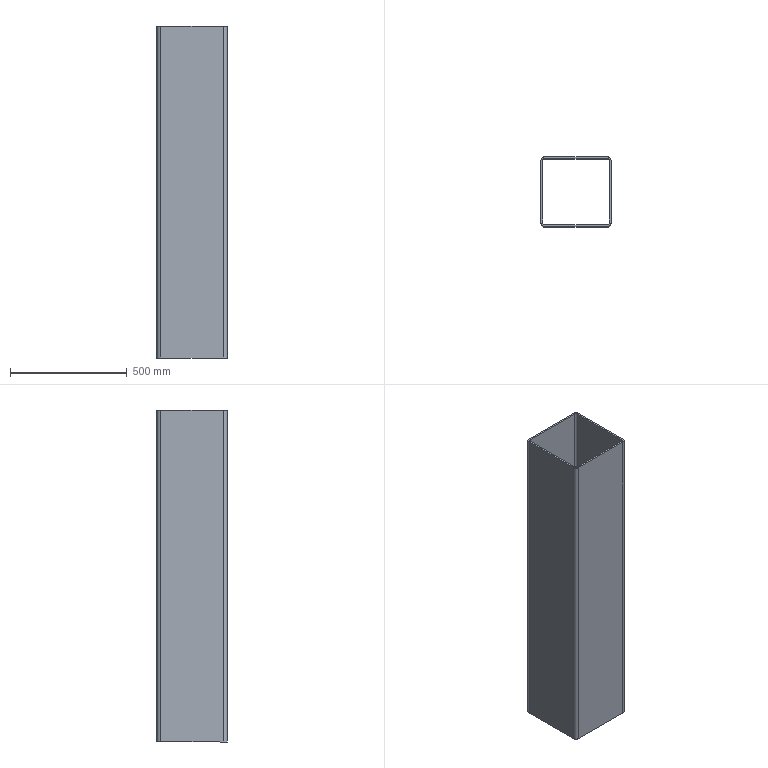Component | SolidWorks | TrolleyLeg-1_300 x 300 x 8-1200-1 | 1 solid | 18 faces | box 300 x 300 x 1420 mm | volume 13034444 mm3 | plane 10 | cylinder 8 | commonest cylinder face diameters 32 x4 16 x4 | material Plain Carbon Steel
build123d program:
from build123d import *

# Parameters (mm, degrees)
BOSS_EXTRUDE1_DEPTH = 1420


with BuildPart() as part:
    # Sketch1 → Boss-Extrude1 (new body)
    with BuildSketch(Plane.XY):
        with BuildLine():
            Line((-134, -150), (134, -150))
            ThreePointArc((134, -150), (145.314, -145.314), (150, -134))
            Line((150, -134), (150, 134))
            ThreePointArc((150, 134), (145.314, 145.314), (134, 150))
            Line((134, 150), (-134, 150))
            ThreePointArc((-134, 150), (-145.314, 145.314), (-150, 134))
            Line((-150, 134), (-150, -134))
            ThreePointArc((-150, -134), (-145.314, -145.314), (-134, -150))
        make_face()
        with BuildLine():
            Line((-134, -142), (134, -142))
            ThreePointArc((134, -142), (139.657, -139.657), (142, -134))
            Line((142, -134), (142, 134))
            ThreePointArc((142, 134), (139.657, 139.657), (134, 142))
            Line((134, 142), (-134, 142))
            ThreePointArc((-134, 142), (-139.657, 139.657), (-142, 134))
            Line((-142, 134), (-142, -134))
            ThreePointArc((-142, -134), (-139.657, -139.657), (-134, -142))
        make_face(mode=Mode.SUBTRACT)
    extrude(amount=BOSS_EXTRUDE1_DEPTH)


solid = part.part

# Placed as in the assembly
solid = solid.moved(Location((-2662.199, 1921.323, 3245.973), (0, 0, 0)))
STEP:
#1=COLOUR_RGB('',0.7922,0.8196,0.9333);
#2=FILL_AREA_STYLE_COLOUR('',#1);
#3=FILL_AREA_STYLE('',(#2));
#4=SURFACE_STYLE_FILL_AREA(#3);
#5=SURFACE_SIDE_STYLE('',(#4));
#6=SURFACE_STYLE_USAGE(.BOTH.,#5);
#7=PRESENTATION_STYLE_ASSIGNMENT((#6));
#8=CARTESIAN_POINT('',(-110.717,80.918,127.794));
#9=VERTEX_POINT('',#8);
#10=CARTESIAN_POINT('',(-110.087,81.548,127.794));
#11=VERTEX_POINT('',#10);
#12=CARTESIAN_POINT('',(-110.087,80.918,127.794));
#13=DIRECTION('',(0.,0.,-1.));
#14=DIRECTION('',(1.,0.,0.));
#15=AXIS2_PLACEMENT_3D('',#12,#13,#14);
#16=CIRCLE('',#15,0.6299);
#17=EDGE_CURVE('',#9,#11,#16,.T.);
#18=ORIENTED_EDGE('',*,*,#17,.T.);
#19=CARTESIAN_POINT('',(-99.535,81.548,127.794));
#20=VERTEX_POINT('',#19);
#21=CARTESIAN_POINT('',(-110.087,81.548,127.794));
#22=DIRECTION('',(1.,0.,0.));
#23=VECTOR('',#22,39.37);
#24=LINE('',#21,#23);
#25=EDGE_CURVE('',#11,#20,#24,.T.);
#26=ORIENTED_EDGE('',*,*,#25,.T.);
#27=CARTESIAN_POINT('',(-98.905,80.918,127.794));
#28=VERTEX_POINT('',#27);
#29=CARTESIAN_POINT('',(-99.535,80.918,127.794));
#30=DIRECTION('',(0.,0.,-1.));
#31=DIRECTION('',(1.,0.,0.));
#32=AXIS2_PLACEMENT_3D('',#29,#30,#31);
#33=CIRCLE('',#32,0.6299);
#34=EDGE_CURVE('',#20,#28,#33,.T.);
#35=ORIENTED_EDGE('',*,*,#34,.T.);
#36=CARTESIAN_POINT('',(-98.905,70.367,127.794));
#37=VERTEX_POINT('',#36);
#38=CARTESIAN_POINT('',(-98.905,70.367,127.794));
#39=DIRECTION('',(0.,1.,0.));
#40=VECTOR('',#39,39.37);
#41=LINE('',#38,#40);
#42=EDGE_CURVE('',#37,#28,#41,.T.);
#43=ORIENTED_EDGE('',*,*,#42,.F.);
#44=CARTESIAN_POINT('',(-99.535,69.737,127.794));
#45=VERTEX_POINT('',#44);
#46=CARTESIAN_POINT('',(-99.535,70.367,127.794));
#47=DIRECTION('',(0.,0.,-1.));
#48=DIRECTION('',(1.,0.,0.));
#49=AXIS2_PLACEMENT_3D('',#46,#47,#48);
#50=CIRCLE('',#49,0.6299);
#51=EDGE_CURVE('',#37,#45,#50,.T.);
#52=ORIENTED_EDGE('',*,*,#51,.T.);
#53=CARTESIAN_POINT('',(-110.087,69.737,127.794));
#54=VERTEX_POINT('',#53);
#55=CARTESIAN_POINT('',(-99.535,69.737,127.794));
#56=DIRECTION('',(-1.,0.,0.));
#57=VECTOR('',#56,39.37);
#58=LINE('',#55,#57);
#59=EDGE_CURVE('',#45,#54,#58,.T.);
#60=ORIENTED_EDGE('',*,*,#59,.T.);
#61=CARTESIAN_POINT('',(-110.717,70.367,127.794));
#62=VERTEX_POINT('',#61);
#63=CARTESIAN_POINT('',(-110.087,70.367,127.794));
#64=DIRECTION('',(0.,0.,-1.));
#65=DIRECTION('',(1.,0.,0.));
#66=AXIS2_PLACEMENT_3D('',#63,#64,#65);
#67=CIRCLE('',#66,0.6299);
#68=EDGE_CURVE('',#54,#62,#67,.T.);
#69=ORIENTED_EDGE('',*,*,#68,.T.);
#70=CARTESIAN_POINT('',(-110.717,80.918,127.794));
#71=DIRECTION('',(0.,-1.,-0.));
#72=VECTOR('',#71,39.37);
#73=LINE('',#70,#72);
#74=EDGE_CURVE('',#9,#62,#73,.T.);
#75=ORIENTED_EDGE('',*,*,#74,.F.);
#76=EDGE_LOOP('',(#18,#26,#35,#43,#52,#60,#69,#75));
#77=FACE_OUTER_BOUND('',#76,.T.);
#78=CARTESIAN_POINT('',(-110.087,81.233,127.794));
#79=VERTEX_POINT('',#78);
#80=CARTESIAN_POINT('',(-99.535,81.233,127.794));
#81=VERTEX_POINT('',#80);
#82=CARTESIAN_POINT('',(-110.087,81.233,127.794));
#83=DIRECTION('',(1.,0.,0.));
#84=VECTOR('',#83,39.37);
#85=LINE('',#82,#84);
#86=EDGE_CURVE('',#79,#81,#85,.T.);
#87=ORIENTED_EDGE('',*,*,#86,.F.);
#88=CARTESIAN_POINT('',(-110.402,80.918,127.794));
#89=VERTEX_POINT('',#88);
#90=CARTESIAN_POINT('',(-110.087,80.918,127.794));
#91=DIRECTION('',(0.,0.,-1.));
#92=DIRECTION('',(1.,0.,0.));
#93=AXIS2_PLACEMENT_3D('',#90,#91,#92);
#94=CIRCLE('',#93,0.315);
#95=EDGE_CURVE('',#89,#79,#94,.T.);
#96=ORIENTED_EDGE('',*,*,#95,.F.);
#97=CARTESIAN_POINT('',(-110.402,70.367,127.794));
#98=VERTEX_POINT('',#97);
#99=CARTESIAN_POINT('',(-110.402,80.918,127.794));
#100=DIRECTION('',(0.,-1.,-0.));
#101=VECTOR('',#100,39.37);
#102=LINE('',#99,#101);
#103=EDGE_CURVE('',#89,#98,#102,.T.);
#104=ORIENTED_EDGE('',*,*,#103,.T.);
#105=CARTESIAN_POINT('',(-110.087,70.052,127.794));
#106=VERTEX_POINT('',#105);
#107=CARTESIAN_POINT('',(-110.087,70.367,127.794));
#108=DIRECTION('',(0.,0.,-1.));
#109=DIRECTION('',(1.,0.,0.));
#110=AXIS2_PLACEMENT_3D('',#107,#108,#109);
#111=CIRCLE('',#110,0.315);
#112=EDGE_CURVE('',#106,#98,#111,.T.);
#113=ORIENTED_EDGE('',*,*,#112,.F.);
#114=CARTESIAN_POINT('',(-99.535,70.052,127.794));
#115=VERTEX_POINT('',#114);
#116=CARTESIAN_POINT('',(-99.535,70.052,127.794));
#117=DIRECTION('',(-1.,0.,0.));
#118=VECTOR('',#117,39.37);
#119=LINE('',#116,#118);
#120=EDGE_CURVE('',#115,#106,#119,.T.);
#121=ORIENTED_EDGE('',*,*,#120,.F.);
#122=CARTESIAN_POINT('',(-99.22,70.367,127.794));
#123=VERTEX_POINT('',#122);
#124=CARTESIAN_POINT('',(-99.535,70.367,127.794));
#125=DIRECTION('',(0.,0.,-1.));
#126=DIRECTION('',(1.,0.,0.));
#127=AXIS2_PLACEMENT_3D('',#124,#125,#126);
#128=CIRCLE('',#127,0.315);
#129=EDGE_CURVE('',#123,#115,#128,.T.);
#130=ORIENTED_EDGE('',*,*,#129,.F.);
#131=CARTESIAN_POINT('',(-99.22,80.918,127.794));
#132=VERTEX_POINT('',#131);
#133=CARTESIAN_POINT('',(-99.22,70.367,127.794));
#134=DIRECTION('',(0.,1.,0.));
#135=VECTOR('',#134,39.37);
#136=LINE('',#133,#135);
#137=EDGE_CURVE('',#123,#132,#136,.T.);
#138=ORIENTED_EDGE('',*,*,#137,.T.);
#139=CARTESIAN_POINT('',(-99.535,80.918,127.794));
#140=DIRECTION('',(0.,0.,-1.));
#141=DIRECTION('',(1.,0.,0.));
#142=AXIS2_PLACEMENT_3D('',#139,#140,#141);
#143=CIRCLE('',#142,0.315);
#144=EDGE_CURVE('',#81,#132,#143,.T.);
#145=ORIENTED_EDGE('',*,*,#144,.F.);
#146=EDGE_LOOP('',(#87,#96,#104,#113,#121,#130,#138,#145));
#147=FACE_BOUND('',#146,.T.);
#148=CARTESIAN_POINT('',(-110.087,80.918,127.794));
#149=DIRECTION('',(0.,0.,-1.));
#150=DIRECTION('',(1.,0.,0.));
#151=AXIS2_PLACEMENT_3D('',#148,#149,#150);
#152=PLANE('',#151);
#153=ADVANCED_FACE('',(#77,#147),#152,.T.);
#154=CARTESIAN_POINT('',(-110.717,80.918,183.7));
#155=VERTEX_POINT('',#154);
#156=CARTESIAN_POINT('',(-110.087,81.548,183.7));
#157=VERTEX_POINT('',#156);
#158=CARTESIAN_POINT('',(-110.087,80.918,183.7));
#159=DIRECTION('',(0.,0.,-1.));
#160=DIRECTION('',(1.,0.,0.));
#161=AXIS2_PLACEMENT_3D('',#158,#159,#160);
#162=CIRCLE('',#161,0.6299);
#163=EDGE_CURVE('',#155,#157,#162,.T.);
#164=ORIENTED_EDGE('',*,*,#163,.F.);
#165=CARTESIAN_POINT('',(-110.717,70.367,183.7));
#166=VERTEX_POINT('',#165);
#167=CARTESIAN_POINT('',(-110.717,80.918,183.7));
#168=DIRECTION('',(0.,-1.,-0.));
#169=VECTOR('',#168,39.37);
#170=LINE('',#167,#169);
#171=EDGE_CURVE('',#155,#166,#170,.T.);
#172=ORIENTED_EDGE('',*,*,#171,.T.);
#173=CARTESIAN_POINT('',(-110.087,69.737,183.7));
#174=VERTEX_POINT('',#173);
#175=CARTESIAN_POINT('',(-110.087,70.367,183.7));
#176=DIRECTION('',(0.,0.,-1.));
#177=DIRECTION('',(1.,0.,0.));
#178=AXIS2_PLACEMENT_3D('',#175,#176,#177);
#179=CIRCLE('',#178,0.6299);
#180=EDGE_CURVE('',#174,#166,#179,.T.);
#181=ORIENTED_EDGE('',*,*,#180,.F.);
#182=CARTESIAN_POINT('',(-99.535,69.737,183.7));
#183=VERTEX_POINT('',#182);
#184=CARTESIAN_POINT('',(-99.535,69.737,183.7));
#185=DIRECTION('',(-1.,0.,0.));
#186=VECTOR('',#185,39.37);
#187=LINE('',#184,#186);
#188=EDGE_CURVE('',#183,#174,#187,.T.);
#189=ORIENTED_EDGE('',*,*,#188,.F.);
#190=CARTESIAN_POINT('',(-98.905,70.367,183.7));
#191=VERTEX_POINT('',#190);
#192=CARTESIAN_POINT('',(-99.535,70.367,183.7));
#193=DIRECTION('',(0.,0.,-1.));
#194=DIRECTION('',(1.,0.,0.));
#195=AXIS2_PLACEMENT_3D('',#192,#193,#194);
#196=CIRCLE('',#195,0.6299);
#197=EDGE_CURVE('',#191,#183,#196,.T.);
#198=ORIENTED_EDGE('',*,*,#197,.F.);
#199=CARTESIAN_POINT('',(-98.905,80.918,183.7));
#200=VERTEX_POINT('',#199);
#201=CARTESIAN_POINT('',(-98.905,70.367,183.7));
#202=DIRECTION('',(0.,1.,0.));
#203=VECTOR('',#202,39.37);
#204=LINE('',#201,#203);
#205=EDGE_CURVE('',#191,#200,#204,.T.);
#206=ORIENTED_EDGE('',*,*,#205,.T.);
#207=CARTESIAN_POINT('',(-99.535,81.548,183.7));
#208=VERTEX_POINT('',#207);
#209=CARTESIAN_POINT('',(-99.535,80.918,183.7));
#210=DIRECTION('',(0.,0.,-1.));
#211=DIRECTION('',(1.,0.,0.));
#212=AXIS2_PLACEMENT_3D('',#209,#210,#211);
#213=CIRCLE('',#212,0.6299);
#214=EDGE_CURVE('',#208,#200,#213,.T.);
#215=ORIENTED_EDGE('',*,*,#214,.F.);
#216=CARTESIAN_POINT('',(-110.087,81.548,183.7));
#217=DIRECTION('',(1.,0.,0.));
#218=VECTOR('',#217,39.37);
#219=LINE('',#216,#218);
#220=EDGE_CURVE('',#157,#208,#219,.T.);
#221=ORIENTED_EDGE('',*,*,#220,.F.);
#222=EDGE_LOOP('',(#164,#172,#181,#189,#198,#206,#215,#221));
#223=FACE_OUTER_BOUND('',#222,.T.);
#224=CARTESIAN_POINT('',(-110.402,80.918,183.7));
#225=VERTEX_POINT('',#224);
#226=CARTESIAN_POINT('',(-110.087,81.233,183.7));
#227=VERTEX_POINT('',#226);
#228=CARTESIAN_POINT('',(-110.087,80.918,183.7));
#229=DIRECTION('',(0.,0.,-1.));
#230=DIRECTION('',(1.,0.,0.));
#231=AXIS2_PLACEMENT_3D('',#228,#229,#230);
#232=CIRCLE('',#231,0.315);
#233=EDGE_CURVE('',#225,#227,#232,.T.);
#234=ORIENTED_EDGE('',*,*,#233,.T.);
#235=CARTESIAN_POINT('',(-99.535,81.233,183.7));
#236=VERTEX_POINT('',#235);
#237=CARTESIAN_POINT('',(-110.087,81.233,183.7));
#238=DIRECTION('',(1.,0.,0.));
#239=VECTOR('',#238,39.37);
#240=LINE('',#237,#239);
#241=EDGE_CURVE('',#227,#236,#240,.T.);
#242=ORIENTED_EDGE('',*,*,#241,.T.);
#243=CARTESIAN_POINT('',(-99.22,80.918,183.7));
#244=VERTEX_POINT('',#243);
#245=CARTESIAN_POINT('',(-99.535,80.918,183.7));
#246=DIRECTION('',(0.,0.,-1.));
#247=DIRECTION('',(1.,0.,0.));
#248=AXIS2_PLACEMENT_3D('',#245,#246,#247);
#249=CIRCLE('',#248,0.315);
#250=EDGE_CURVE('',#236,#244,#249,.T.);
#251=ORIENTED_EDGE('',*,*,#250,.T.);
#252=CARTESIAN_POINT('',(-99.22,70.367,183.7));
#253=VERTEX_POINT('',#252);
#254=CARTESIAN_POINT('',(-99.22,70.367,183.7));
#255=DIRECTION('',(0.,1.,0.));
#256=VECTOR('',#255,39.37);
#257=LINE('',#254,#256);
#258=EDGE_CURVE('',#253,#244,#257,.T.);
#259=ORIENTED_EDGE('',*,*,#258,.F.);
#260=CARTESIAN_POINT('',(-99.535,70.052,183.7));
#261=VERTEX_POINT('',#260);
#262=CARTESIAN_POINT('',(-99.535,70.367,183.7));
#263=DIRECTION('',(0.,0.,-1.));
#264=DIRECTION('',(1.,0.,0.));
#265=AXIS2_PLACEMENT_3D('',#262,#263,#264);
#266=CIRCLE('',#265,0.315);
#267=EDGE_CURVE('',#253,#261,#266,.T.);
#268=ORIENTED_EDGE('',*,*,#267,.T.);
#269=CARTESIAN_POINT('',(-110.087,70.052,183.7));
#270=VERTEX_POINT('',#269);
#271=CARTESIAN_POINT('',(-99.535,70.052,183.7));
#272=DIRECTION('',(-1.,0.,0.));
#273=VECTOR('',#272,39.37);
#274=LINE('',#271,#273);
#275=EDGE_CURVE('',#261,#270,#274,.T.);
#276=ORIENTED_EDGE('',*,*,#275,.T.);
#277=CARTESIAN_POINT('',(-110.402,70.367,183.7));
#278=VERTEX_POINT('',#277);
#279=CARTESIAN_POINT('',(-110.087,70.367,183.7));
#280=DIRECTION('',(0.,0.,-1.));
#281=DIRECTION('',(1.,0.,0.));
#282=AXIS2_PLACEMENT_3D('',#279,#280,#281);
#283=CIRCLE('',#282,0.315);
#284=EDGE_CURVE('',#270,#278,#283,.T.);
#285=ORIENTED_EDGE('',*,*,#284,.T.);
#286=CARTESIAN_POINT('',(-110.402,80.918,183.7));
#287=DIRECTION('',(0.,-1.,-0.));
#288=VECTOR('',#287,39.37);
#289=LINE('',#286,#288);
#290=EDGE_CURVE('',#225,#278,#289,.T.);
#291=ORIENTED_EDGE('',*,*,#290,.F.);
#292=EDGE_LOOP('',(#234,#242,#251,#259,#268,#276,#285,#291));
#293=FACE_BOUND('',#292,.T.);
#294=CARTESIAN_POINT('',(-110.087,80.918,183.7));
#295=DIRECTION('',(0.,0.,-1.));
#296=DIRECTION('',(1.,0.,0.));
#297=AXIS2_PLACEMENT_3D('',#294,#295,#296);
#298=PLANE('',#297);
#299=ADVANCED_FACE('',(#223,#293),#298,.F.);
#300=ORIENTED_EDGE('',*,*,#163,.T.);
#301=CARTESIAN_POINT('',(-110.087,81.548,127.794));
#302=DIRECTION('',(0.,-0.,1.));
#303=VECTOR('',#302,39.37);
#304=LINE('',#301,#303);
#305=EDGE_CURVE('',#11,#157,#304,.T.);
#306=ORIENTED_EDGE('',*,*,#305,.F.);
#307=ORIENTED_EDGE('',*,*,#17,.F.);
#308=CARTESIAN_POINT('',(-110.717,80.918,127.794));
#309=DIRECTION('',(0.,-0.,1.));
#310=VECTOR('',#309,39.37);
#311=LINE('',#308,#310);
#312=EDGE_CURVE('',#9,#155,#311,.T.);
#313=ORIENTED_EDGE('',*,*,#312,.T.);
#314=EDGE_LOOP('',(#300,#306,#307,#313));
#315=FACE_OUTER_BOUND('',#314,.T.);
#316=CARTESIAN_POINT('',(-110.087,80.918,127.794));
#317=DIRECTION('',(0.,-0.,1.));
#318=DIRECTION('',(-1.,0.,0.));
#319=AXIS2_PLACEMENT_3D('',#316,#317,#318);
#320=CYLINDRICAL_SURFACE('',#319,0.6299);
#321=ADVANCED_FACE('',(#315),#320,.T.);
#322=ORIENTED_EDGE('',*,*,#220,.T.);
#323=CARTESIAN_POINT('',(-99.535,81.548,127.794));
#324=DIRECTION('',(0.,-0.,1.));
#325=VECTOR('',#324,39.37);
#326=LINE('',#323,#325);
#327=EDGE_CURVE('',#20,#208,#326,.T.);
#328=ORIENTED_EDGE('',*,*,#327,.F.);
#329=ORIENTED_EDGE('',*,*,#25,.F.);
#330=ORIENTED_EDGE('',*,*,#305,.T.);
#331=EDGE_LOOP('',(#322,#328,#329,#330));
#332=FACE_OUTER_BOUND('',#331,.T.);
#333=CARTESIAN_POINT('',(-110.087,81.548,127.794));
#334=DIRECTION('',(0.,-1.,-0.));
#335=DIRECTION('',(0.,0.,-1.));
#336=AXIS2_PLACEMENT_3D('',#333,#334,#335);
#337=PLANE('',#336);
#338=ADVANCED_FACE('',(#332),#337,.F.);
#339=ORIENTED_EDGE('',*,*,#214,.T.);
#340=CARTESIAN_POINT('',(-98.905,80.918,127.794));
#341=DIRECTION('',(0.,-0.,1.));
#342=VECTOR('',#341,39.37);
#343=LINE('',#340,#342);
#344=EDGE_CURVE('',#28,#200,#343,.T.);
#345=ORIENTED_EDGE('',*,*,#344,.F.);
#346=ORIENTED_EDGE('',*,*,#34,.F.);
#347=ORIENTED_EDGE('',*,*,#327,.T.);
#348=EDGE_LOOP('',(#339,#345,#346,#347));
#349=FACE_OUTER_BOUND('',#348,.T.);
#350=CARTESIAN_POINT('',(-99.535,80.918,127.794));
#351=DIRECTION('',(0.,-0.,1.));
#352=DIRECTION('',(-1.,0.,0.));
#353=AXIS2_PLACEMENT_3D('',#350,#351,#352);
#354=CYLINDRICAL_SURFACE('',#353,0.6299);
#355=ADVANCED_FACE('',(#349),#354,.T.);
#356=ORIENTED_EDGE('',*,*,#205,.F.);
#357=CARTESIAN_POINT('',(-98.905,70.367,127.794));
#358=DIRECTION('',(0.,-0.,1.));
#359=VECTOR('',#358,39.37);
#360=LINE('',#357,#359);
#361=EDGE_CURVE('',#37,#191,#360,.T.);
#362=ORIENTED_EDGE('',*,*,#361,.F.);
#363=ORIENTED_EDGE('',*,*,#42,.T.);
#364=ORIENTED_EDGE('',*,*,#344,.T.);
#365=EDGE_LOOP('',(#356,#362,#363,#364));
#366=FACE_OUTER_BOUND('',#365,.T.);
#367=CARTESIAN_POINT('',(-98.905,70.367,127.794));
#368=DIRECTION('',(1.,0.,0.));
#369=DIRECTION('',(0.,-0.,1.));
#370=AXIS2_PLACEMENT_3D('',#367,#368,#369);
#371=PLANE('',#370);
#372=ADVANCED_FACE('',(#366),#371,.T.);
#373=ORIENTED_EDGE('',*,*,#197,.T.);
#374=CARTESIAN_POINT('',(-99.535,69.737,127.794));
#375=DIRECTION('',(0.,-0.,1.));
#376=VECTOR('',#375,39.37);
#377=LINE('',#374,#376);
#378=EDGE_CURVE('',#45,#183,#377,.T.);
#379=ORIENTED_EDGE('',*,*,#378,.F.);
#380=ORIENTED_EDGE('',*,*,#51,.F.);
#381=ORIENTED_EDGE('',*,*,#361,.T.);
#382=EDGE_LOOP('',(#373,#379,#380,#381));
#383=FACE_OUTER_BOUND('',#382,.T.);
#384=CARTESIAN_POINT('',(-99.535,70.367,127.794));
#385=DIRECTION('',(0.,-0.,1.));
#386=DIRECTION('',(-1.,0.,0.));
#387=AXIS2_PLACEMENT_3D('',#384,#385,#386);
#388=CYLINDRICAL_SURFACE('',#387,0.6299);
#389=ADVANCED_FACE('',(#383),#388,.T.);
#390=ORIENTED_EDGE('',*,*,#188,.T.);
#391=CARTESIAN_POINT('',(-110.087,69.737,127.794));
#392=DIRECTION('',(0.,-0.,1.));
#393=VECTOR('',#392,39.37);
#394=LINE('',#391,#393);
#395=EDGE_CURVE('',#54,#174,#394,.T.);
#396=ORIENTED_EDGE('',*,*,#395,.F.);
#397=ORIENTED_EDGE('',*,*,#59,.F.);
#398=ORIENTED_EDGE('',*,*,#378,.T.);
#399=EDGE_LOOP('',(#390,#396,#397,#398));
#400=FACE_OUTER_BOUND('',#399,.T.);
#401=CARTESIAN_POINT('',(-99.535,69.737,127.794));
#402=DIRECTION('',(0.,1.,0.));
#403=DIRECTION('',(0.,-0.,1.));
#404=AXIS2_PLACEMENT_3D('',#401,#402,#403);
#405=PLANE('',#404);
#406=ADVANCED_FACE('',(#400),#405,.F.);
#407=ORIENTED_EDGE('',*,*,#180,.T.);
#408=CARTESIAN_POINT('',(-110.717,70.367,127.794));
#409=DIRECTION('',(0.,-0.,1.));
#410=VECTOR('',#409,39.37);
#411=LINE('',#408,#410);
#412=EDGE_CURVE('',#62,#166,#411,.T.);
#413=ORIENTED_EDGE('',*,*,#412,.F.);
#414=ORIENTED_EDGE('',*,*,#68,.F.);
#415=ORIENTED_EDGE('',*,*,#395,.T.);
#416=EDGE_LOOP('',(#407,#413,#414,#415));
#417=FACE_OUTER_BOUND('',#416,.T.);
#418=CARTESIAN_POINT('',(-110.087,70.367,127.794));
#419=DIRECTION('',(0.,-0.,1.));
#420=DIRECTION('',(-1.,0.,0.));
#421=AXIS2_PLACEMENT_3D('',#418,#419,#420);
#422=CYLINDRICAL_SURFACE('',#421,0.6299);
#423=ADVANCED_FACE('',(#417),#422,.T.);
#424=ORIENTED_EDGE('',*,*,#171,.F.);
#425=ORIENTED_EDGE('',*,*,#312,.F.);
#426=ORIENTED_EDGE('',*,*,#74,.T.);
#427=ORIENTED_EDGE('',*,*,#412,.T.);
#428=EDGE_LOOP('',(#424,#425,#426,#427));
#429=FACE_OUTER_BOUND('',#428,.T.);
#430=CARTESIAN_POINT('',(-110.717,80.918,127.794));
#431=DIRECTION('',(-1.,0.,0.));
#432=DIRECTION('',(0.,0.,-1.));
#433=AXIS2_PLACEMENT_3D('',#430,#431,#432);
#434=PLANE('',#433);
#435=ADVANCED_FACE('',(#429),#434,.T.);
#436=ORIENTED_EDGE('',*,*,#233,.F.);
#437=CARTESIAN_POINT('',(-110.402,80.918,127.794));
#438=DIRECTION('',(0.,-0.,1.));
#439=VECTOR('',#438,39.37);
#440=LINE('',#437,#439);
#441=EDGE_CURVE('',#89,#225,#440,.T.);
#442=ORIENTED_EDGE('',*,*,#441,.F.);
#443=ORIENTED_EDGE('',*,*,#95,.T.);
#444=CARTESIAN_POINT('',(-110.087,81.233,127.794));
#445=DIRECTION('',(0.,-0.,1.));
#446=VECTOR('',#445,39.37);
#447=LINE('',#444,#446);
#448=EDGE_CURVE('',#79,#227,#447,.T.);
#449=ORIENTED_EDGE('',*,*,#448,.T.);
#450=EDGE_LOOP('',(#436,#442,#443,#449));
#451=FACE_OUTER_BOUND('',#450,.T.);
#452=CARTESIAN_POINT('',(-110.087,80.918,127.794));
#453=DIRECTION('',(0.,-0.,1.));
#454=DIRECTION('',(-1.,0.,0.));
#455=AXIS2_PLACEMENT_3D('',#452,#453,#454);
#456=CYLINDRICAL_SURFACE('',#455,0.315);
#457=ADVANCED_FACE('',(#451),#456,.F.);
#458=ORIENTED_EDGE('',*,*,#241,.F.);
#459=ORIENTED_EDGE('',*,*,#448,.F.);
#460=ORIENTED_EDGE('',*,*,#86,.T.);
#461=CARTESIAN_POINT('',(-99.535,81.233,127.794));
#462=DIRECTION('',(0.,-0.,1.));
#463=VECTOR('',#462,39.37);
#464=LINE('',#461,#463);
#465=EDGE_CURVE('',#81,#236,#464,.T.);
#466=ORIENTED_EDGE('',*,*,#465,.T.);
#467=EDGE_LOOP('',(#458,#459,#460,#466));
#468=FACE_OUTER_BOUND('',#467,.T.);
#469=CARTESIAN_POINT('',(-110.087,81.233,127.794));
#470=DIRECTION('',(0.,-1.,-0.));
#471=DIRECTION('',(0.,0.,-1.));
#472=AXIS2_PLACEMENT_3D('',#469,#470,#471);
#473=PLANE('',#472);
#474=ADVANCED_FACE('',(#468),#473,.T.);
#475=ORIENTED_EDGE('',*,*,#250,.F.);
#476=ORIENTED_EDGE('',*,*,#465,.F.);
#477=ORIENTED_EDGE('',*,*,#144,.T.);
#478=CARTESIAN_POINT('',(-99.22,80.918,127.794));
#479=DIRECTION('',(0.,-0.,1.));
#480=VECTOR('',#479,39.37);
#481=LINE('',#478,#480);
#482=EDGE_CURVE('',#132,#244,#481,.T.);
#483=ORIENTED_EDGE('',*,*,#482,.T.);
#484=EDGE_LOOP('',(#475,#476,#477,#483));
#485=FACE_OUTER_BOUND('',#484,.T.);
#486=CARTESIAN_POINT('',(-99.535,80.918,127.794));
#487=DIRECTION('',(0.,-0.,1.));
#488=DIRECTION('',(-1.,0.,0.));
#489=AXIS2_PLACEMENT_3D('',#486,#487,#488);
#490=CYLINDRICAL_SURFACE('',#489,0.315);
#491=ADVANCED_FACE('',(#485),#490,.F.);
#492=ORIENTED_EDGE('',*,*,#258,.T.);
#493=ORIENTED_EDGE('',*,*,#482,.F.);
#494=ORIENTED_EDGE('',*,*,#137,.F.);
#495=CARTESIAN_POINT('',(-99.22,70.367,127.794));
#496=DIRECTION('',(0.,-0.,1.));
#497=VECTOR('',#496,39.37);
#498=LINE('',#495,#497);
#499=EDGE_CURVE('',#123,#253,#498,.T.);
#500=ORIENTED_EDGE('',*,*,#499,.T.);
#501=EDGE_LOOP('',(#492,#493,#494,#500));
#502=FACE_OUTER_BOUND('',#501,.T.);
#503=CARTESIAN_POINT('',(-99.22,70.367,127.794));
#504=DIRECTION('',(1.,0.,0.));
#505=DIRECTION('',(0.,-0.,1.));
#506=AXIS2_PLACEMENT_3D('',#503,#504,#505);
#507=PLANE('',#506);
#508=ADVANCED_FACE('',(#502),#507,.F.);
#509=ORIENTED_EDGE('',*,*,#267,.F.);
#510=ORIENTED_EDGE('',*,*,#499,.F.);
#511=ORIENTED_EDGE('',*,*,#129,.T.);
#512=CARTESIAN_POINT('',(-99.535,70.052,127.794));
#513=DIRECTION('',(0.,-0.,1.));
#514=VECTOR('',#513,39.37);
#515=LINE('',#512,#514);
#516=EDGE_CURVE('',#115,#261,#515,.T.);
#517=ORIENTED_EDGE('',*,*,#516,.T.);
#518=EDGE_LOOP('',(#509,#510,#511,#517));
#519=FACE_OUTER_BOUND('',#518,.T.);
#520=CARTESIAN_POINT('',(-99.535,70.367,127.794));
#521=DIRECTION('',(0.,-0.,1.));
#522=DIRECTION('',(-1.,0.,0.));
#523=AXIS2_PLACEMENT_3D('',#520,#521,#522);
#524=CYLINDRICAL_SURFACE('',#523,0.315);
#525=ADVANCED_FACE('',(#519),#524,.F.);
#526=ORIENTED_EDGE('',*,*,#275,.F.);
#527=ORIENTED_EDGE('',*,*,#516,.F.);
#528=ORIENTED_EDGE('',*,*,#120,.T.);
#529=CARTESIAN_POINT('',(-110.087,70.052,127.794));
#530=DIRECTION('',(0.,-0.,1.));
#531=VECTOR('',#530,39.37);
#532=LINE('',#529,#531);
#533=EDGE_CURVE('',#106,#270,#532,.T.);
#534=ORIENTED_EDGE('',*,*,#533,.T.);
#535=EDGE_LOOP('',(#526,#527,#528,#534));
#536=FACE_OUTER_BOUND('',#535,.T.);
#537=CARTESIAN_POINT('',(-99.535,70.052,127.794));
#538=DIRECTION('',(0.,1.,0.));
#539=DIRECTION('',(0.,-0.,1.));
#540=AXIS2_PLACEMENT_3D('',#537,#538,#539);
#541=PLANE('',#540);
#542=ADVANCED_FACE('',(#536),#541,.T.);
#543=ORIENTED_EDGE('',*,*,#284,.F.);
#544=ORIENTED_EDGE('',*,*,#533,.F.);
#545=ORIENTED_EDGE('',*,*,#112,.T.);
#546=CARTESIAN_POINT('',(-110.402,70.367,127.794));
#547=DIRECTION('',(0.,-0.,1.));
#548=VECTOR('',#547,39.37);
#549=LINE('',#546,#548);
#550=EDGE_CURVE('',#98,#278,#549,.T.);
#551=ORIENTED_EDGE('',*,*,#550,.T.);
#552=EDGE_LOOP('',(#543,#544,#545,#551));
#553=FACE_OUTER_BOUND('',#552,.T.);
#554=CARTESIAN_POINT('',(-110.087,70.367,127.794));
#555=DIRECTION('',(0.,-0.,1.));
#556=DIRECTION('',(-1.,0.,0.));
#557=AXIS2_PLACEMENT_3D('',#554,#555,#556);
#558=CYLINDRICAL_SURFACE('',#557,0.315);
#559=ADVANCED_FACE('',(#553),#558,.F.);
#560=ORIENTED_EDGE('',*,*,#290,.T.);
#561=ORIENTED_EDGE('',*,*,#550,.F.);
#562=ORIENTED_EDGE('',*,*,#103,.F.);
#563=ORIENTED_EDGE('',*,*,#441,.T.);
#564=EDGE_LOOP('',(#560,#561,#562,#563));
#565=FACE_OUTER_BOUND('',#564,.T.);
#566=CARTESIAN_POINT('',(-110.402,80.918,127.794));
#567=DIRECTION('',(-1.,0.,0.));
#568=DIRECTION('',(0.,0.,-1.));
#569=AXIS2_PLACEMENT_3D('',#566,#567,#568);
#570=PLANE('',#569);
#571=ADVANCED_FACE('',(#565),#570,.F.);
#572=CLOSED_SHELL('',(#153,#299,#321,#338,#355,#372,#389,#406,#423,#435,#457,#474,#491,#508,#525,#542,#559,#571));
#573=MANIFOLD_SOLID_BREP('',#572);
#574=STYLED_ITEM('',(#7),#573);
#575=(LENGTH_UNIT()NAMED_UNIT(*)SI_UNIT($,.METRE.));
#576=LENGTH_MEASURE_WITH_UNIT(LENGTH_MEASURE(0.0254),#575);
#577=DIMENSIONAL_EXPONENTS(1.,0.,0.,0.,0.,0.,0.);
#578=(CONVERSION_BASED_UNIT('',#576)LENGTH_UNIT()NAMED_UNIT(#577));
#579=UNCERTAINTY_MEASURE_WITH_UNIT(LENGTH_MEASURE(0.00001),#578,'','');
#580=(NAMED_UNIT(*)PLANE_ANGLE_UNIT()SI_UNIT($,.RADIAN.));
#581=(NAMED_UNIT(*)SI_UNIT($,.STERADIAN.)SOLID_ANGLE_UNIT());
#582=(GEOMETRIC_REPRESENTATION_CONTEXT(3)GLOBAL_UNCERTAINTY_ASSIGNED_CONTEXT((#579))GLOBAL_UNIT_ASSIGNED_CONTEXT((#578,#580,#581))REPRESENTATION_CONTEXT('',''));
#583=MECHANICAL_DESIGN_GEOMETRIC_PRESENTATION_REPRESENTATION('',(#574),#582);
#584=CARTESIAN_POINT('',(0.,0.,0.));
#585=DIRECTION('',(0.,0.,1.));
#586=DIRECTION('',(1.,0.,0.));
#587=AXIS2_PLACEMENT_3D('',#584,#585,#586);
#588=(LENGTH_UNIT()NAMED_UNIT(*)SI_UNIT($,.METRE.));
#589=LENGTH_MEASURE_WITH_UNIT(LENGTH_MEASURE(0.0254),#588);
#590=DIMENSIONAL_EXPONENTS(1.,0.,0.,0.,0.,0.,0.);
#591=(CONVERSION_BASED_UNIT('',#589)LENGTH_UNIT()NAMED_UNIT(#590));
#592=UNCERTAINTY_MEASURE_WITH_UNIT(LENGTH_MEASURE(0.00001),#591,'','');
#593=(NAMED_UNIT(*)PLANE_ANGLE_UNIT()SI_UNIT($,.RADIAN.));
#594=(NAMED_UNIT(*)SI_UNIT($,.STERADIAN.)SOLID_ANGLE_UNIT());
#595=(GEOMETRIC_REPRESENTATION_CONTEXT(3)GLOBAL_UNCERTAINTY_ASSIGNED_CONTEXT((#592))GLOBAL_UNIT_ASSIGNED_CONTEXT((#591,#593,#594))REPRESENTATION_CONTEXT('',''));
#596=ADVANCED_BREP_SHAPE_REPRESENTATION('',(#573,#587),#595);
#597=PRESENTATION_LAYER_ASSIGNMENT('','',(#574));